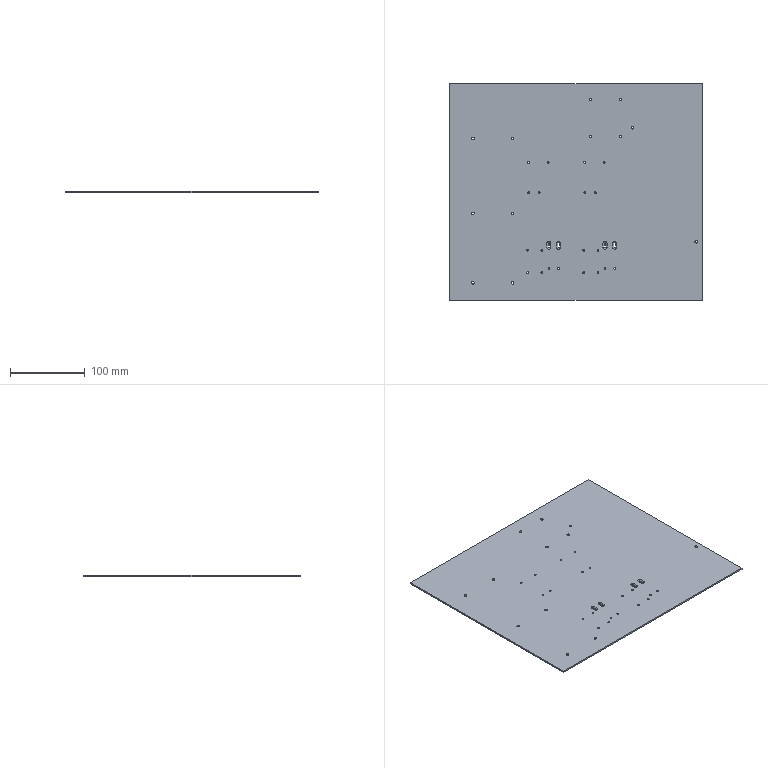CAM job | Mastercam | mm | 3 operations | part box 338 x 290 x 2
1. Contour (Ramp) | 2 - 2 平铣刀
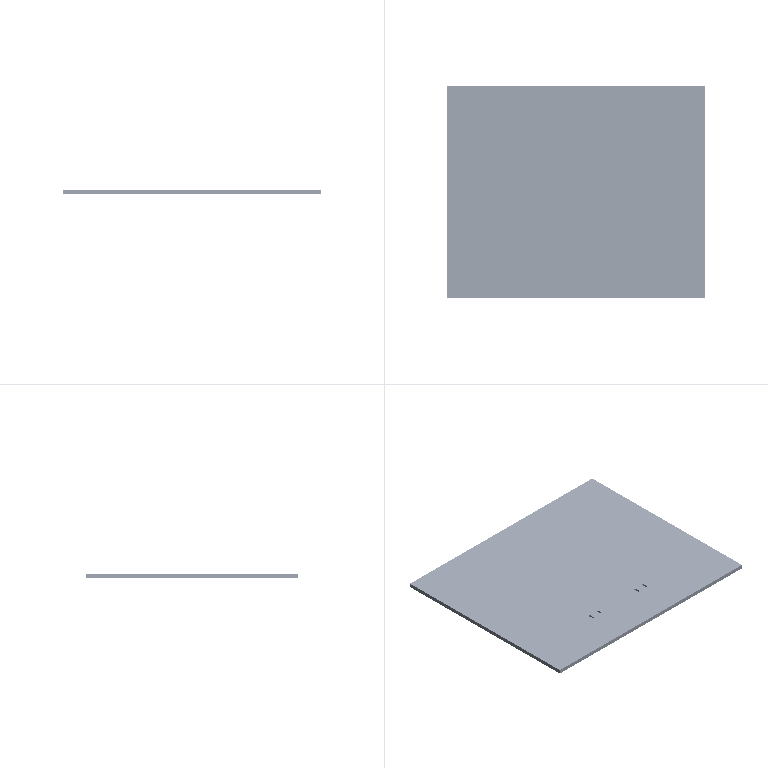2. Drill/Counterbore | 7 - 6 倒角刀
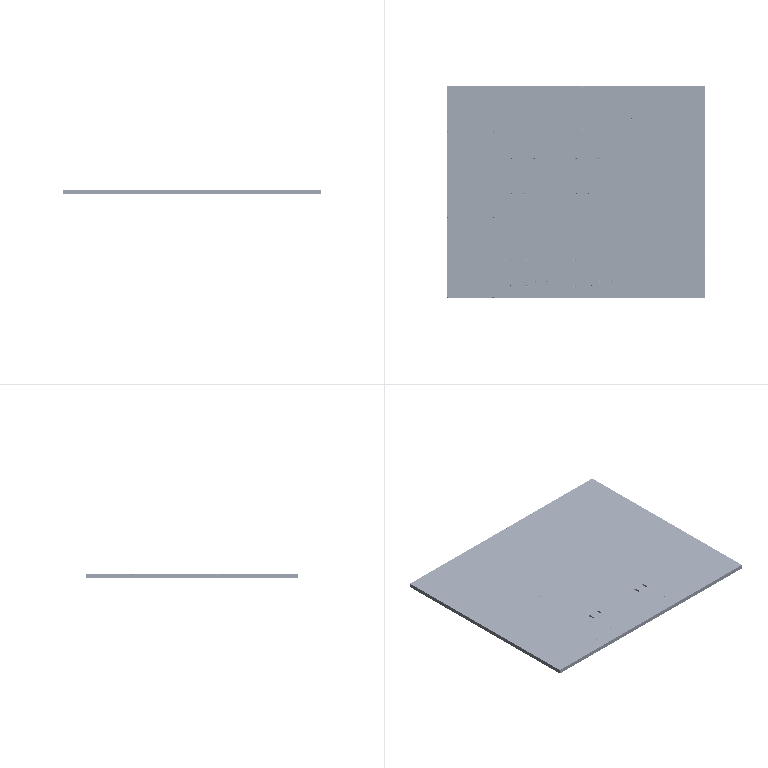3. Contour (2D chamfer) | 7 - 6 倒角刀